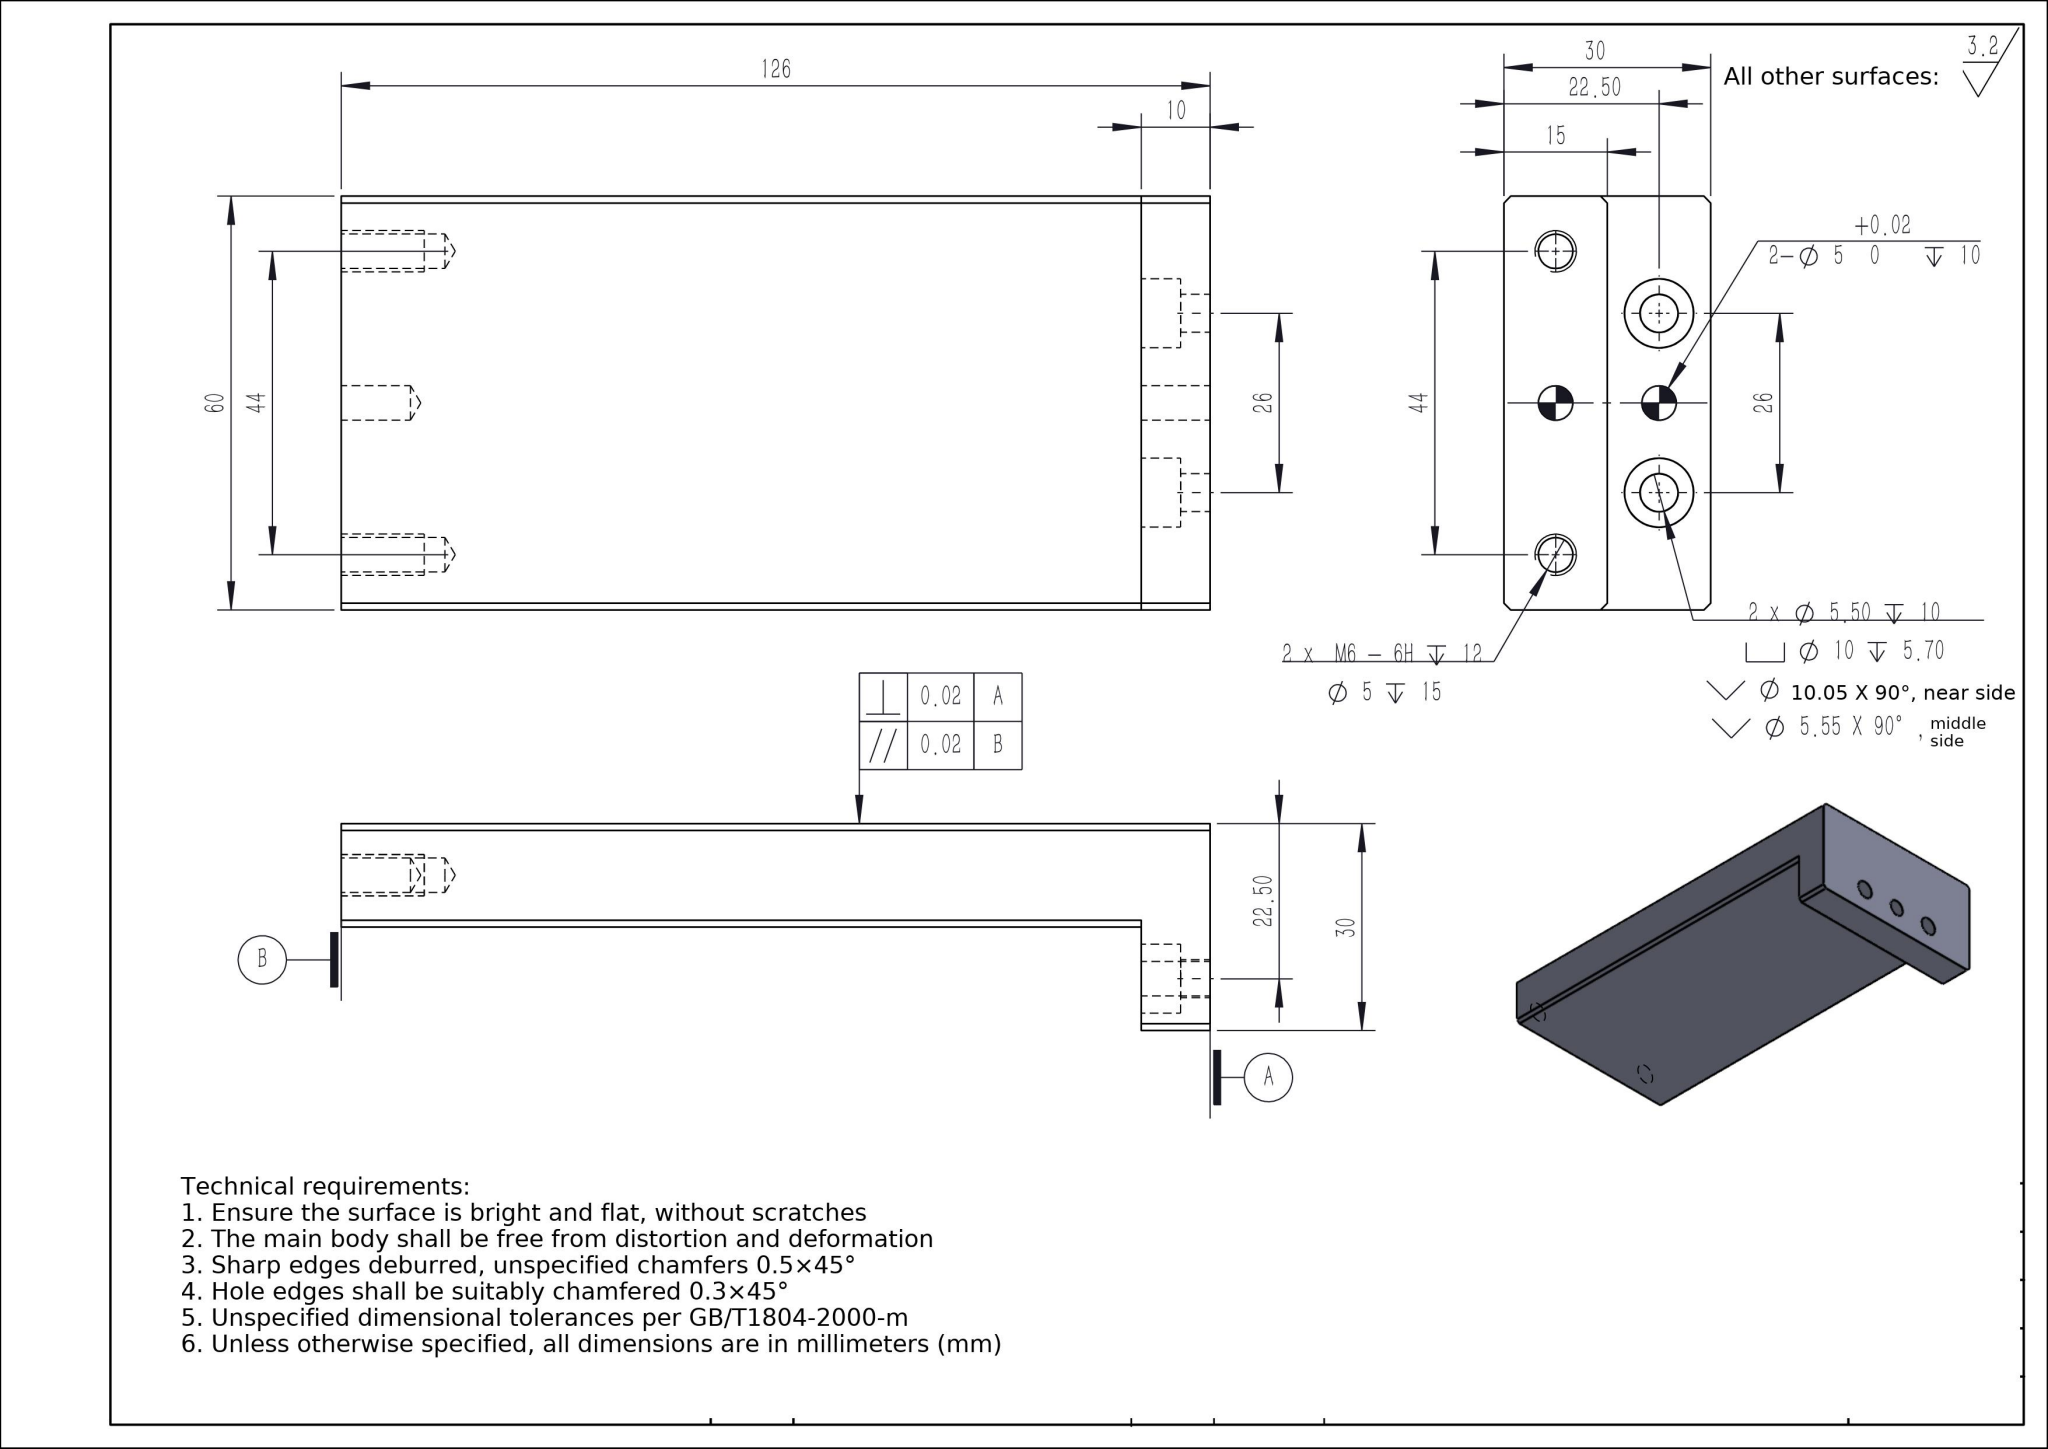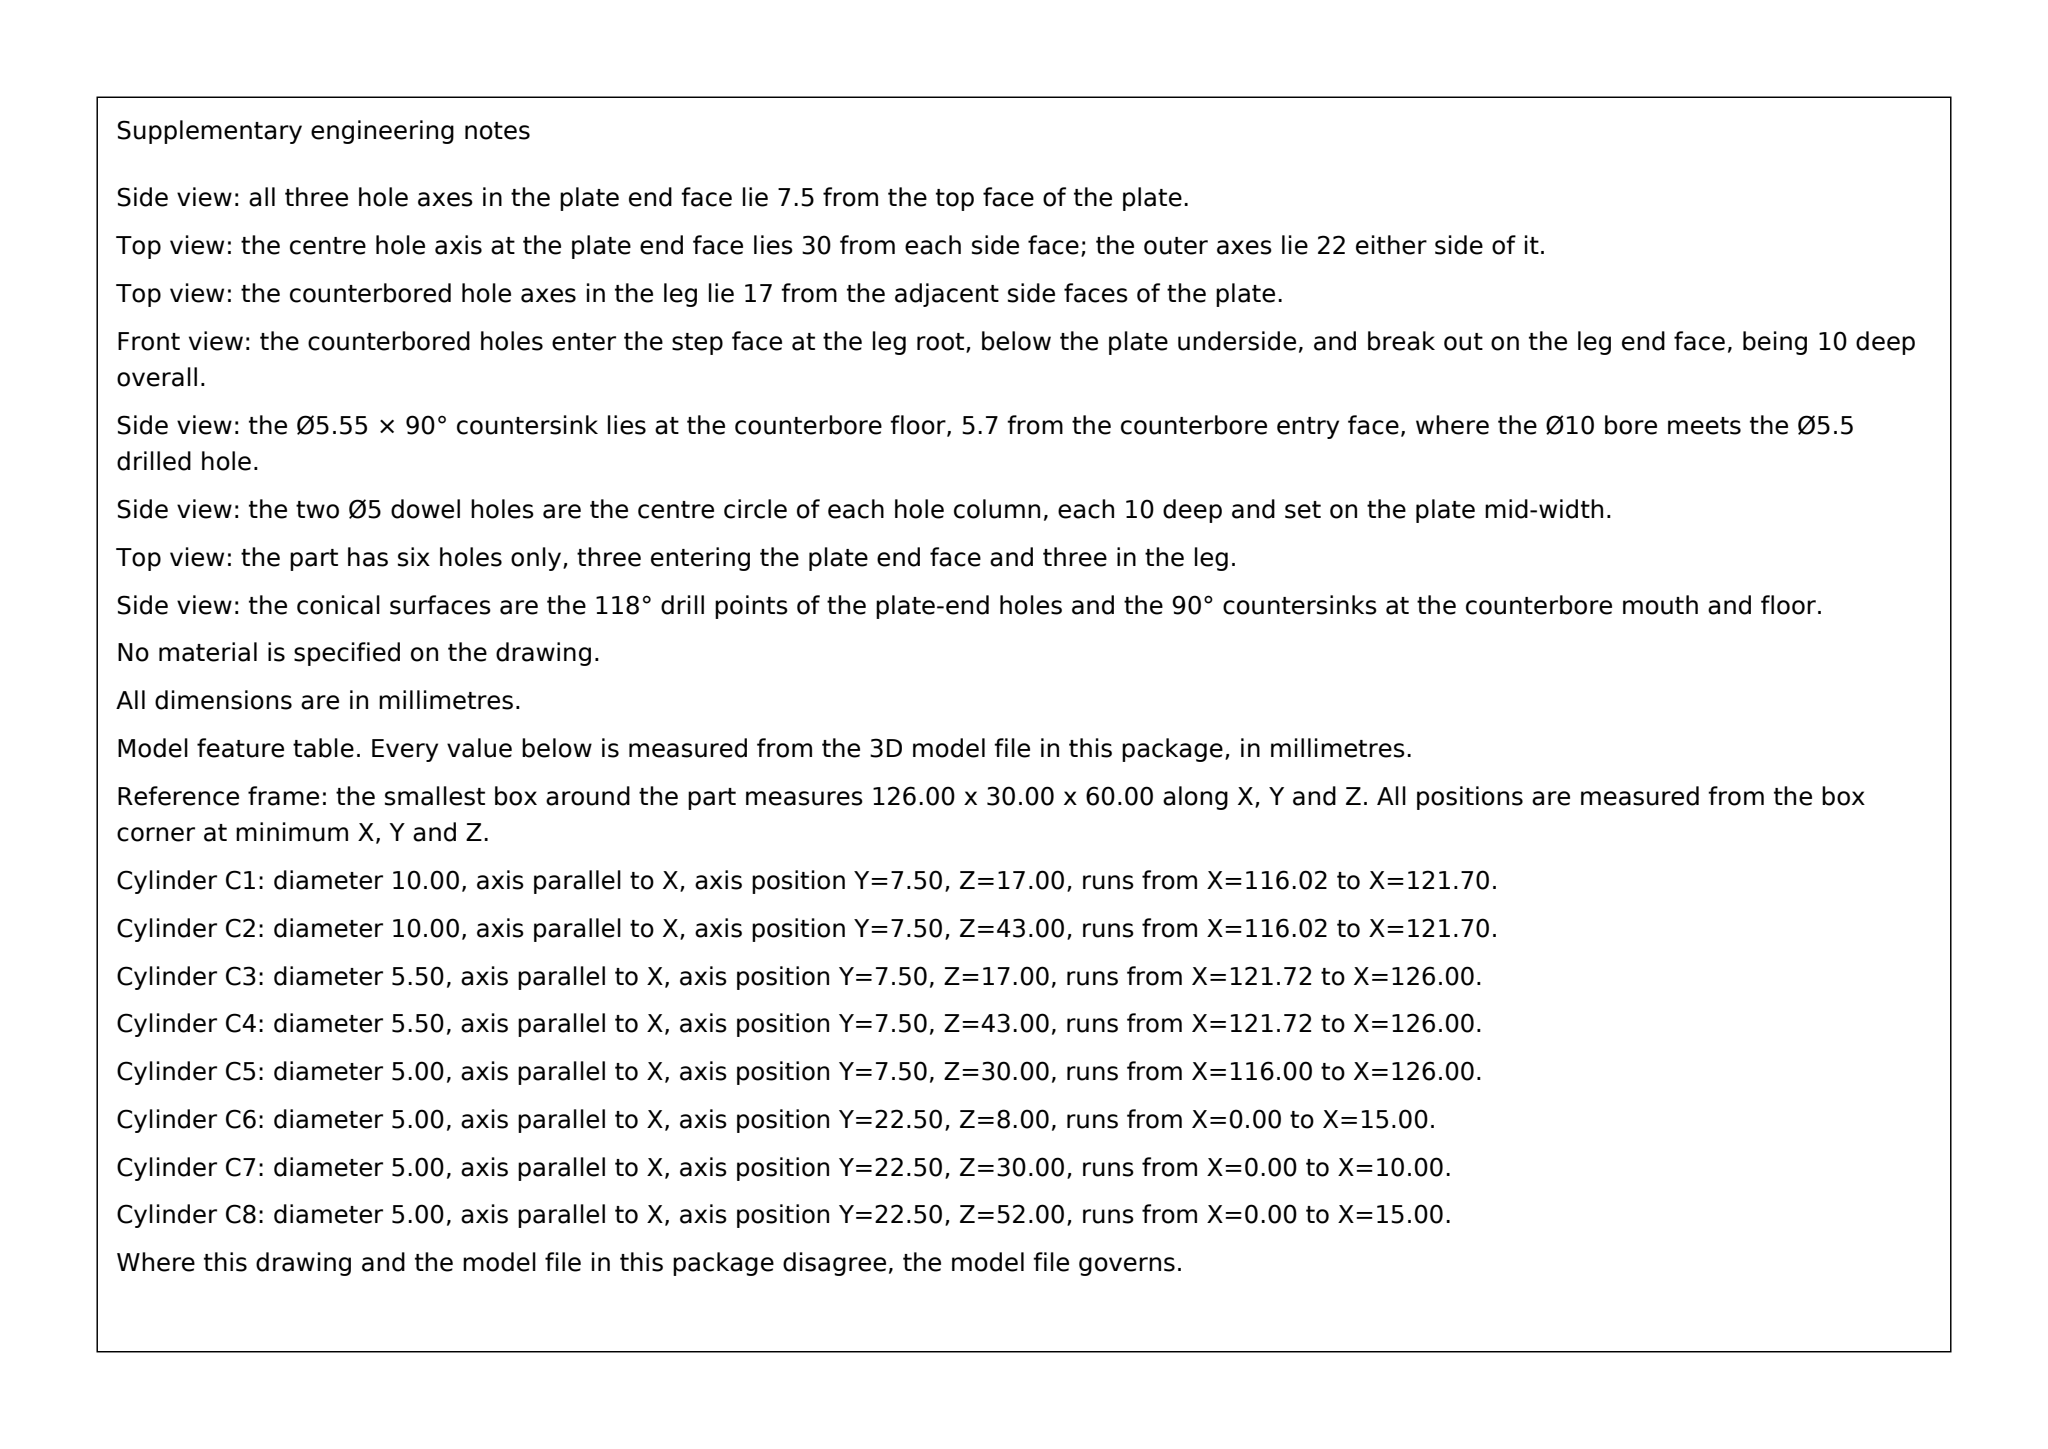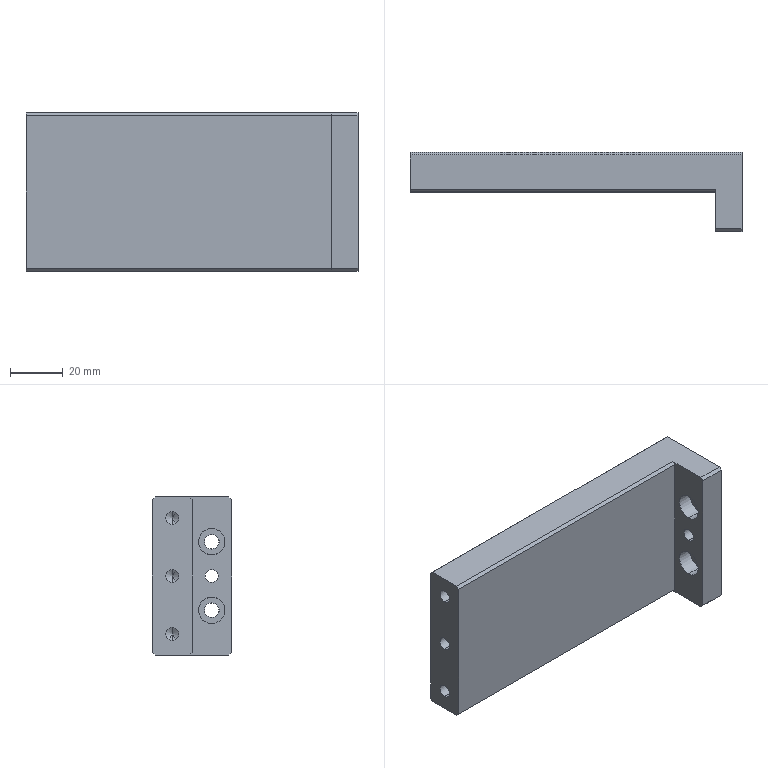Part | SolidWorks | mm | 1 solid | 46 faces | box 126 x 30 x 60 mm | volume 120037 mm3 | cylinder 16 | plane 16 | cone 14 | commonest cylinder face diameters 5 x8 10 x4 5.5 x4
Drawing notes:
2x M6-6H DP 12, Ø5 pilot DP 15: 22.5 from btm face, 22 ea side of 60 CL | from the solid: Ø5 x15 deep bores, axis x, at y=22.5, z=8.0 & 52.0 (bbox 126x30x60; z CL=30, 44 apart)
2-Ø5 +0.02 DP 10 on 60 CL: 7.5 & 22.5 from btm face | from the solid: Ø5 x10 deep bores, axis x, at (y=7.5, z=30.0) and (y=22.5, z=30.0)
build123d program:
from build123d import *

# Parameters (mm, degrees)
SKETCH1_W                                 = 126
SKETCH1_H                                 = 60
BOSS_EXTRUDE1_DEPTH                       = 15
CHAMFER1_SIZE                             = 1
M6_TAPPED_HOLE1_D                         = 5
M6_TAPPED_HOLE1_DEPTH                     = 15
M6_TAPPED_HOLE1_TIP                       = 1.502
SIZE_MM_DOWEL_PIN_HOLE1_D                 = 5
SIZE_MM_DOWEL_PIN_HOLE1_DEPTH             = 10
SIZE_MM_DOWEL_PIN_HOLE1_TIP               = 1.502
BOSS_EXTRUDE2_DEPTH                       = 15
BOSS_EXTRUDE2_DEPTH_BACK                  = 10
SKETCH7_W                                 = 10
SKETCH7_H                                 = 60
HOLE_SIZE_ACCORDING_TO_HEXAGON_SO_2_COUNT = 2
HOLE_SIZE_ACCORDING_TO_HEXAGON_SO_2_PITCH = 26
SIZE_MM_DOWEL_PIN_HOLE2_D                 = 5
SIZE_MM_DOWEL_PIN_HOLE2_DEPTH             = 10
SIZE_MM_DOWEL_PIN_HOLE2_TIP               = 1.502
CHAMFER2_SIZE                             = 1


with BuildPart() as part:
    # Sketch1 → Boss-Extrude1 (new body)
    with BuildSketch(Plane(origin=(0, 0, 0), x_dir=(1, 0, 0), z_dir=(0, 1, 0))):
        Rectangle(SKETCH1_W, SKETCH1_H)
    extrude(amount=BOSS_EXTRUDE1_DEPTH)

    # Chamfer1
    chamfer1_edges = [part.edges().sort_by_distance(p)[0] for p in [
        (0, 15, 30),
        (0, 0, 30),
        (0, 0, -30),
        (0, 15, -30),
    ]]
    chamfer(chamfer1_edges, length=CHAMFER1_SIZE)

    # M6 Tapped Hole1
    with Locations(Plane.ZY.offset(63)):
        with Locations((-22, 7.5), (22, 7.5)):
            Hole(M6_TAPPED_HOLE1_D / 2, depth=M6_TAPPED_HOLE1_DEPTH)
            with Locations((0, 0, -(M6_TAPPED_HOLE1_DEPTH + M6_TAPPED_HOLE1_TIP / 2))):  # 118° drill point
                Cone(0, M6_TAPPED_HOLE1_D / 2, M6_TAPPED_HOLE1_TIP, mode=Mode.SUBTRACT)

    # Size mm Dowel Pin Hole1
    with Locations(Plane.ZY.offset(63)):
        with Locations((0, 7.5)):
            Hole(SIZE_MM_DOWEL_PIN_HOLE1_D / 2, depth=SIZE_MM_DOWEL_PIN_HOLE1_DEPTH)
            with Locations((0, 0, -(SIZE_MM_DOWEL_PIN_HOLE1_DEPTH + SIZE_MM_DOWEL_PIN_HOLE1_TIP / 2))):  # 118° drill point
                Cone(0, SIZE_MM_DOWEL_PIN_HOLE1_D / 2, SIZE_MM_DOWEL_PIN_HOLE1_TIP, mode=Mode.SUBTRACT)

    # Sketch7 → Boss-Extrude2 (add, two sides: drawn at the far end of the back side and taken through both)
    with BuildSketch(Plane(origin=(0, 0, 0), x_dir=(-1, 0, 0), z_dir=(0, -1, 0)).offset(-BOSS_EXTRUDE2_DEPTH_BACK)):
        with Locations((-58, 0)):
            Rectangle(SKETCH7_W, SKETCH7_H)
    extrude(amount=BOSS_EXTRUDE2_DEPTH + BOSS_EXTRUDE2_DEPTH_BACK)

    # Sketch8 → Hole Size _ according to_ Hexagon Socket (revolve, cut)
    with BuildSketch(Plane(origin=(53, -7.5, -13), x_dir=(0, 0, 1), z_dir=(0, 1, 0))):
        Polygon((0, 0), (0, 11.652), (2.75, 10), (2.75, 5.725), (2.775, 5.7), (5, 5.7), (5, 0.025), (5.025, 0), align=None)
    hole_size_according_to_hexagon_socket = revolve(axis=Axis((46.65, -7.5, -13), (1, 0, 0)), mode=Mode.SUBTRACT)

    # Hole Size _ according to_ Hexagon So 2: Hole Size _ according to_ Hexagon Socket ×2
    with Locations(*[(0, 0, i * HOLE_SIZE_ACCORDING_TO_HEXAGON_SO_2_PITCH) for i in range(1, HOLE_SIZE_ACCORDING_TO_HEXAGON_SO_2_COUNT)]):
        add(hole_size_according_to_hexagon_socket, mode=Mode.SUBTRACT)

    # Size mm Dowel Pin Hole2
    with Locations(Plane.ZY.offset(-53)):
        with Locations((0, -7.5)):
            Hole(SIZE_MM_DOWEL_PIN_HOLE2_D / 2, depth=SIZE_MM_DOWEL_PIN_HOLE2_DEPTH)
            with Locations((0, 0, -(SIZE_MM_DOWEL_PIN_HOLE2_DEPTH + SIZE_MM_DOWEL_PIN_HOLE2_TIP / 2))):  # 118° drill point
                Cone(0, SIZE_MM_DOWEL_PIN_HOLE2_D / 2, SIZE_MM_DOWEL_PIN_HOLE2_TIP, mode=Mode.SUBTRACT)

    # Chamfer2
    chamfer2_edges = [part.edges().sort_by_distance(p)[0] for p in [
        (58, -15, 30),
        (58, -15, -30),
    ]]
    chamfer(chamfer2_edges, length=CHAMFER2_SIZE)


solid = part.part